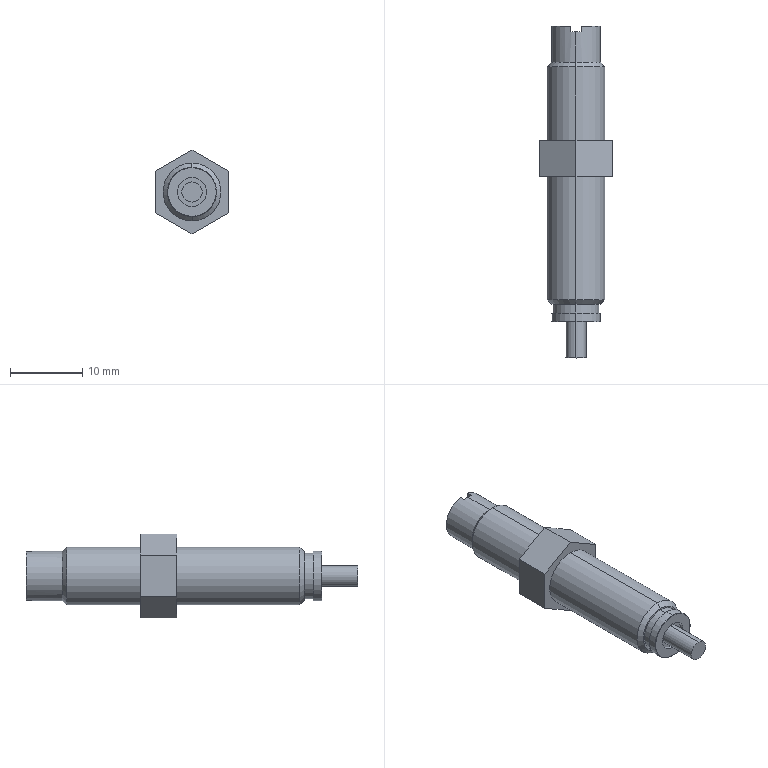Component | SolidWorks | HandlingMechanism-2_1..2659899830.0-1 | 1 solid | 39 faces | volume 2134 mm3 | plane 19 | cylinder 14 | cone 4 | spline 2 | commonest cylinder face diameters 8 x4 6.8 x4 6.3 x2 4 x2 2.8 x2